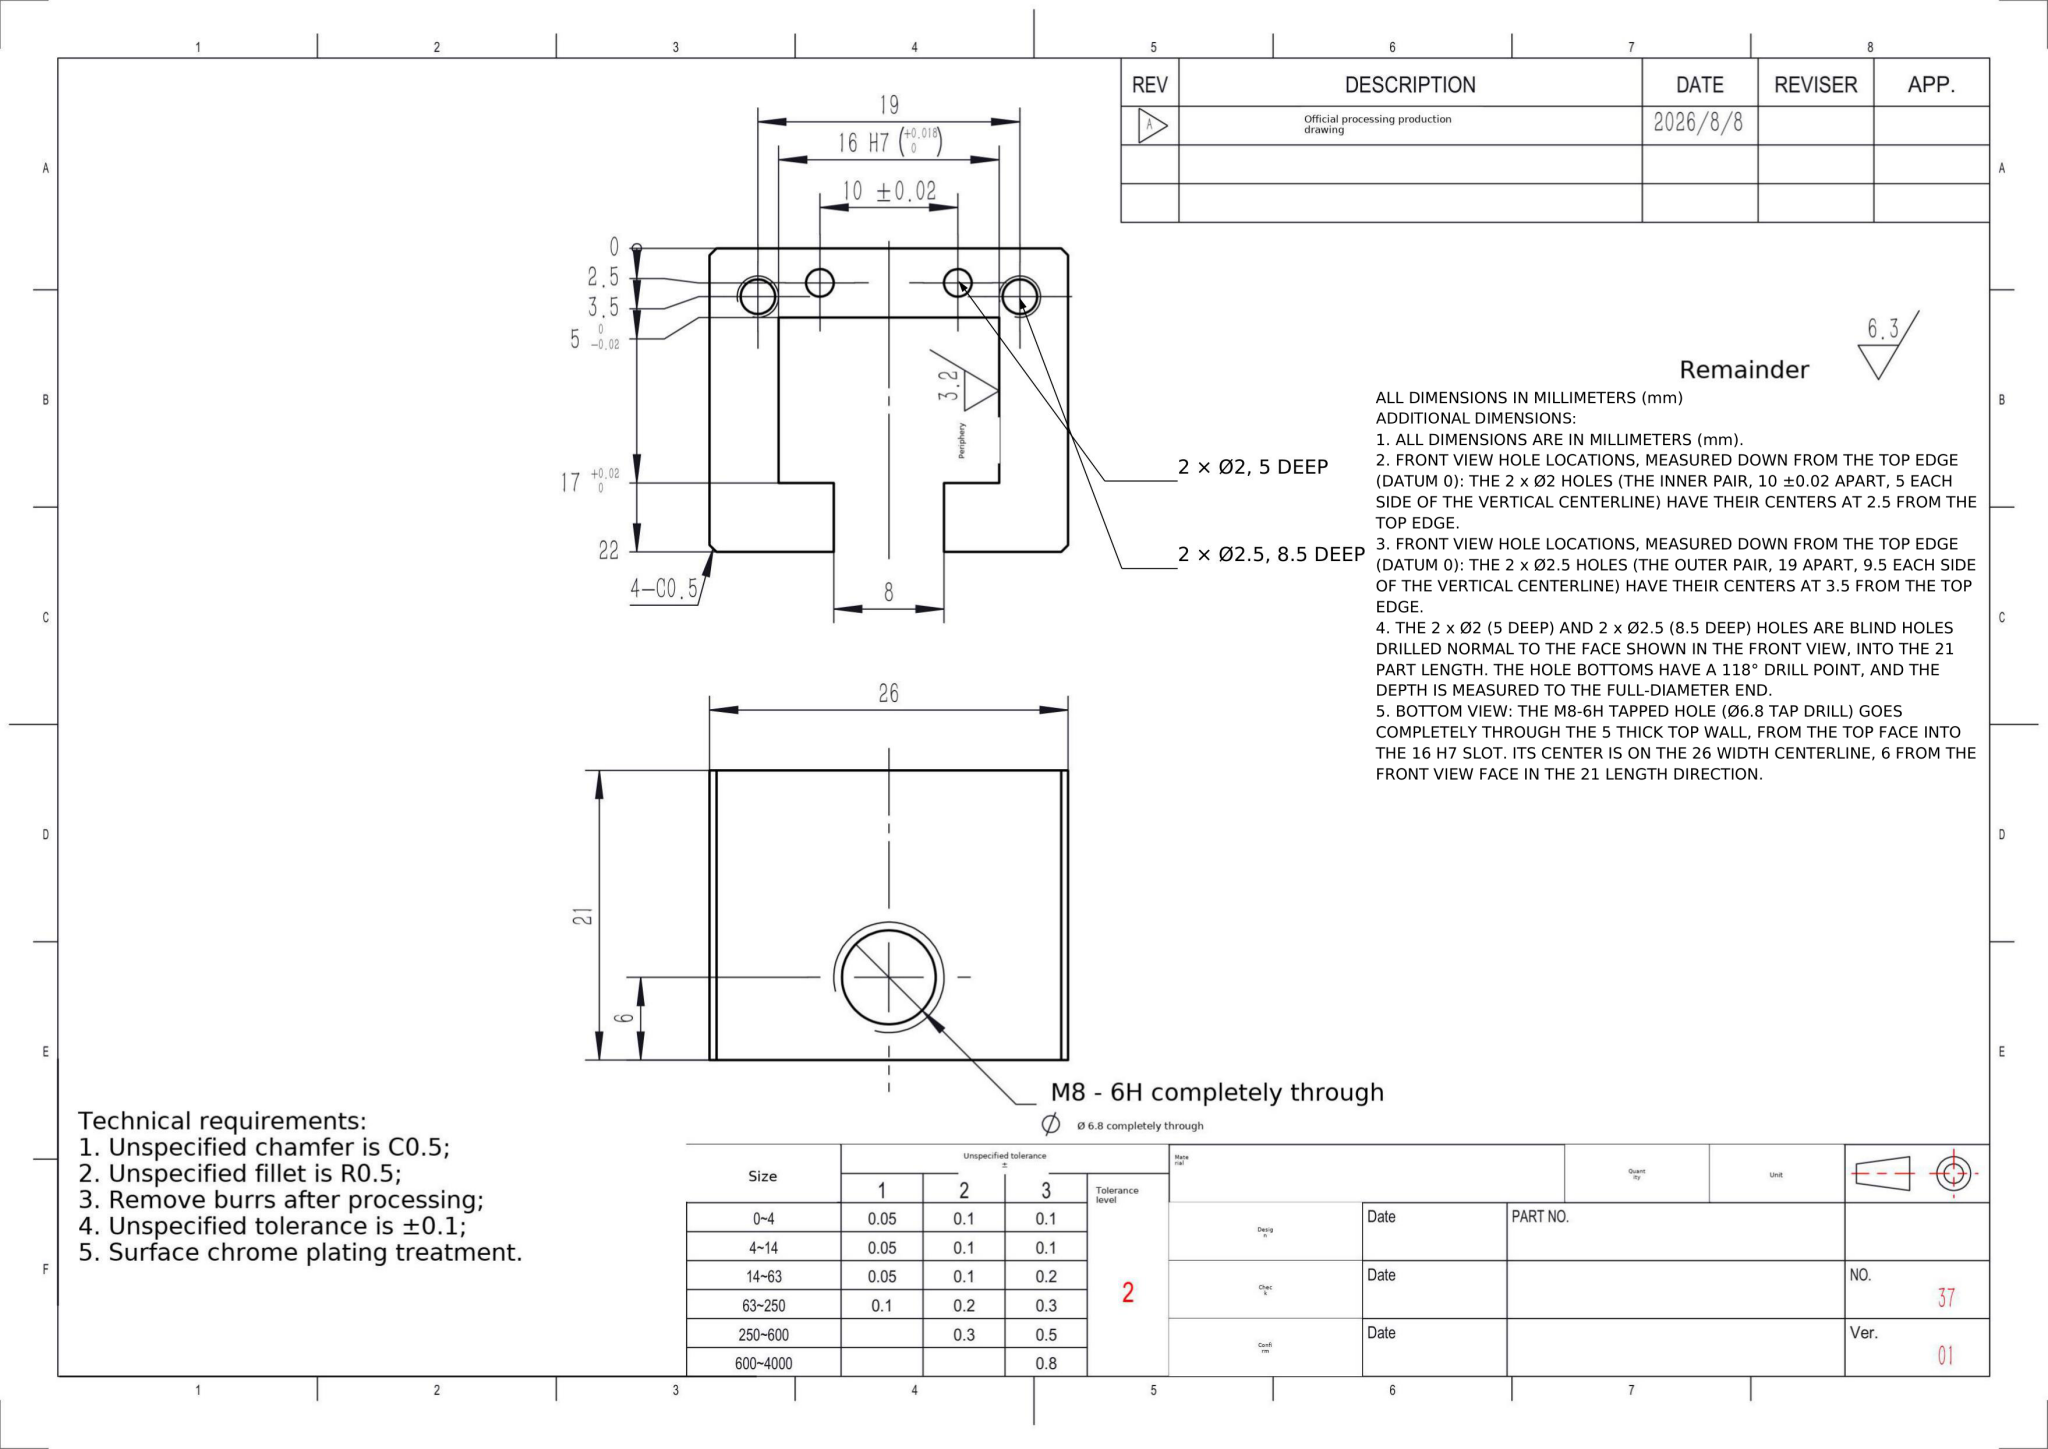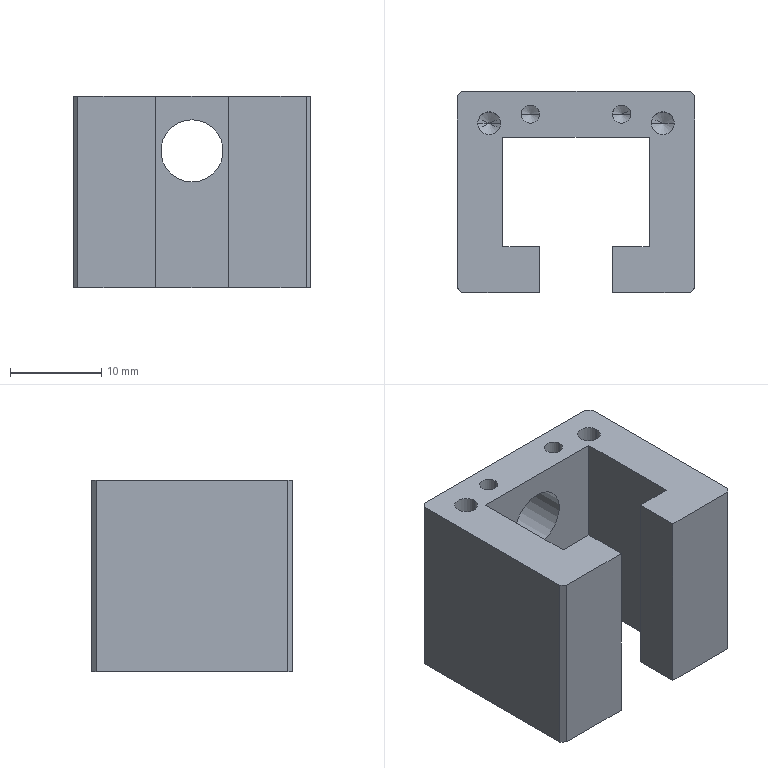Part | NX | mm | Stepped U-Shaped Bearing Mounting Block | 1 solid | 36 faces | box 26 x 22 x 21 mm | volume 6829 mm3 | plane 18 | cylinder 10 | cone 8 | commonest cylinder face diameters 2 x4 2.5 x4 6.8 x2